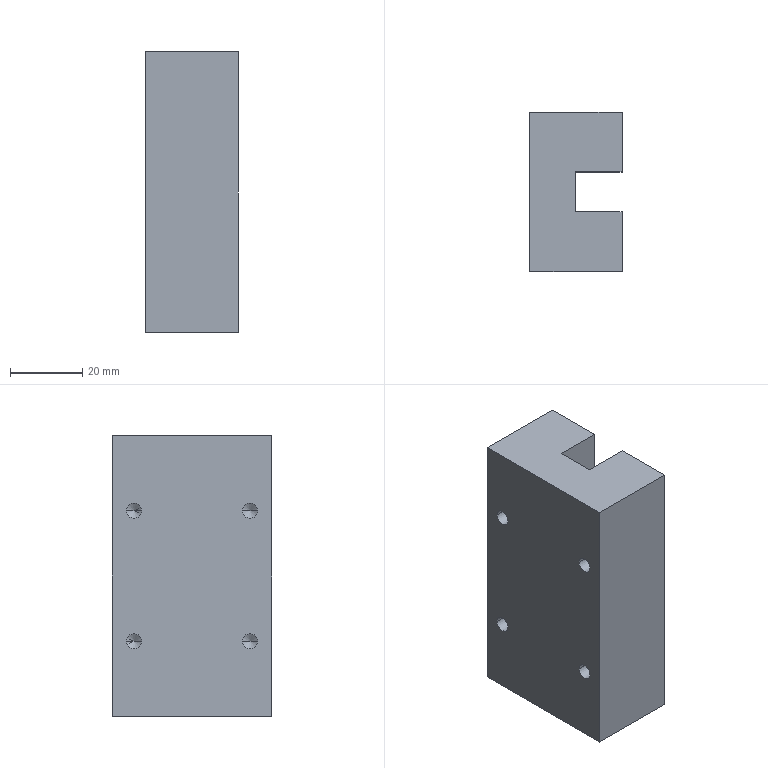Component | SolidWorks | HGH20CASlider-2 | 1 solid | 26 faces | box 25.41 x 44 x 77.5 mm | volume 75261 mm3 | plane 10 | cylinder 8 | cone 8 | commonest cylinder face diameters 4.2 x8
build123d program:
from build123d import *

# Parameters (mm, degrees)
SKETCH1_W             = 44
SKETCH1_H             = 77.5
BOSS_EXTRUDE1_DEPTH   = 25.4
SKETCH2_W             = 11
SKETCH2_H             = 12.9
CUT_EXTRUDE1_DEPTH    = 77.5
M5_TAPPED_HOLE1_D     = 4.2
M5_TAPPED_HOLE1_DEPTH = 6
M5_TAPPED_HOLE1_TIP   = 1.262


with BuildPart() as part:
    # Sketch1 → Boss-Extrude1 (new body)
    with BuildSketch(Plane.XY):
        Rectangle(SKETCH1_W, SKETCH1_H)
    extrude(amount=BOSS_EXTRUDE1_DEPTH)

    # Sketch2 → Cut-Extrude1 (cut)
    with BuildSketch(Plane(origin=(0, 38.75, 0), x_dir=(1, 0, 0), z_dir=(0, 1, 0))):
        with Locations((0, -18.95)):
            Rectangle(SKETCH2_W, SKETCH2_H)
    extrude(amount=-CUT_EXTRUDE1_DEPTH, mode=Mode.SUBTRACT)

    # M5 Tapped Hole1
    with Locations(Plane(origin=(0, 0, 0), x_dir=(-1, 0, 0), z_dir=(0, 0, -1))):
        with Locations((-16, 18), (-16, -18), (16, 18), (16, -18)):
            Hole(M5_TAPPED_HOLE1_D / 2, depth=M5_TAPPED_HOLE1_DEPTH)
            with Locations((0, 0, -(M5_TAPPED_HOLE1_DEPTH + M5_TAPPED_HOLE1_TIP / 2))):  # 118° drill point
                Cone(0, M5_TAPPED_HOLE1_D / 2, M5_TAPPED_HOLE1_TIP, mode=Mode.SUBTRACT)


solid = part.part

# Placed as in the assembly
solid = solid.moved(Location((1956.163, 3833.761, 1079.241), (90, 90, 0)))
STEP:
#1=COLOUR_RGB('',0.7922,0.8196,0.9333);
#2=FILL_AREA_STYLE_COLOUR('',#1);
#3=FILL_AREA_STYLE('',(#2));
#4=SURFACE_STYLE_FILL_AREA(#3);
#5=SURFACE_SIDE_STYLE('',(#4));
#6=SURFACE_STYLE_USAGE(.BOTH.,#5);
#7=PRESENTATION_STYLE_ASSIGNMENT((#6));
#8=CARTESIAN_POINT('',(77.251,150.223,41.781));
#9=VERTEX_POINT('',#8);
#10=CARTESIAN_POINT('',(77.251,150.388,41.781));
#11=VERTEX_POINT('',#10);
#12=CARTESIAN_POINT('',(77.251,150.306,41.781));
#13=DIRECTION('',(-1.,-0.0001552,-0.));
#14=DIRECTION('',(-0.0001552,1.,0.));
#15=AXIS2_PLACEMENT_3D('',#12,#13,#14);
#16=CIRCLE('',#15,0.08268);
#17=EDGE_CURVE('',#9,#11,#16,.T.);
#18=ORIENTED_EDGE('',*,*,#17,.F.);
#19=CARTESIAN_POINT('',(77.014,150.223,41.781));
#20=VERTEX_POINT('',#19);
#21=CARTESIAN_POINT('',(77.014,150.223,41.781));
#22=DIRECTION('',(-1.,-0.0001552,-0.));
#23=VECTOR('',#22,39.37);
#24=LINE('',#21,#23);
#25=EDGE_CURVE('',#9,#20,#24,.T.);
#26=ORIENTED_EDGE('',*,*,#25,.T.);
#27=CARTESIAN_POINT('',(77.014,150.388,41.781));
#28=VERTEX_POINT('',#27);
#29=CARTESIAN_POINT('',(77.014,150.305,41.781));
#30=DIRECTION('',(-1.,-0.0001552,-0.));
#31=DIRECTION('',(-0.0001552,1.,0.));
#32=AXIS2_PLACEMENT_3D('',#29,#30,#31);
#33=CIRCLE('',#32,0.08268);
#34=EDGE_CURVE('',#20,#28,#33,.T.);
#35=ORIENTED_EDGE('',*,*,#34,.T.);
#36=CARTESIAN_POINT('',(77.014,150.388,41.781));
#37=DIRECTION('',(-1.,-0.0001552,-0.));
#38=VECTOR('',#37,39.37);
#39=LINE('',#36,#38);
#40=EDGE_CURVE('',#11,#28,#39,.T.);
#41=ORIENTED_EDGE('',*,*,#40,.F.);
#42=EDGE_LOOP('',(#18,#26,#35,#41));
#43=FACE_OUTER_BOUND('',#42,.T.);
#44=CARTESIAN_POINT('',(77.014,150.305,41.781));
#45=DIRECTION('',(-1.,-0.0001552,-0.));
#46=DIRECTION('',(-0.0001552,1.,0.));
#47=AXIS2_PLACEMENT_3D('',#44,#45,#46);
#48=CYLINDRICAL_SURFACE('',#47,0.08268);
#49=ADVANCED_FACE('',(#43),#48,.F.);
#50=CARTESIAN_POINT('',(77.3,150.306,41.781));
#51=VERTEX_POINT('',#50);
#52=CARTESIAN_POINT('',(77.251,150.388,41.781));
#53=DIRECTION('',(-0.5152,0.8571,-0.));
#54=VECTOR('',#53,39.37);
#55=LINE('',#52,#54);
#56=EDGE_CURVE('',#51,#11,#55,.T.);
#57=ORIENTED_EDGE('',*,*,#56,.F.);
#58=CARTESIAN_POINT('',(77.251,150.223,41.781));
#59=DIRECTION('',(-0.5149,-0.8572,0.));
#60=VECTOR('',#59,39.37);
#61=LINE('',#58,#60);
#62=EDGE_CURVE('',#51,#9,#61,.T.);
#63=ORIENTED_EDGE('',*,*,#62,.T.);
#64=ORIENTED_EDGE('',*,*,#17,.T.);
#65=EDGE_LOOP('',(#57,#63,#64));
#66=FACE_OUTER_BOUND('',#65,.T.);
#67=CARTESIAN_POINT('',(77.251,150.306,41.781));
#68=DIRECTION('',(-1.,-0.0001552,-0.));
#69=DIRECTION('',(-0.0001552,1.,0.));
#70=AXIS2_PLACEMENT_3D('',#67,#68,#69);
#71=CONICAL_SURFACE('',#70,0.08268,1.03);
#72=ADVANCED_FACE('',(#66),#71,.F.);
#73=CARTESIAN_POINT('',(77.251,150.223,43.198));
#74=VERTEX_POINT('',#73);
#75=CARTESIAN_POINT('',(77.251,150.388,43.198));
#76=VERTEX_POINT('',#75);
#77=CARTESIAN_POINT('',(77.251,150.306,43.198));
#78=DIRECTION('',(-1.,-0.0001552,-0.));
#79=DIRECTION('',(-0.0001552,1.,0.));
#80=AXIS2_PLACEMENT_3D('',#77,#78,#79);
#81=CIRCLE('',#80,0.08268);
#82=EDGE_CURVE('',#74,#76,#81,.T.);
#83=ORIENTED_EDGE('',*,*,#82,.F.);
#84=CARTESIAN_POINT('',(77.014,150.223,43.198));
#85=VERTEX_POINT('',#84);
#86=CARTESIAN_POINT('',(77.014,150.223,43.198));
#87=DIRECTION('',(-1.,-0.0001552,-0.));
#88=VECTOR('',#87,39.37);
#89=LINE('',#86,#88);
#90=EDGE_CURVE('',#74,#85,#89,.T.);
#91=ORIENTED_EDGE('',*,*,#90,.T.);
#92=CARTESIAN_POINT('',(77.014,150.388,43.198));
#93=VERTEX_POINT('',#92);
#94=CARTESIAN_POINT('',(77.014,150.305,43.198));
#95=DIRECTION('',(-1.,-0.0001552,-0.));
#96=DIRECTION('',(-0.0001552,1.,0.));
#97=AXIS2_PLACEMENT_3D('',#94,#95,#96);
#98=CIRCLE('',#97,0.08268);
#99=EDGE_CURVE('',#85,#93,#98,.T.);
#100=ORIENTED_EDGE('',*,*,#99,.T.);
#101=CARTESIAN_POINT('',(77.014,150.388,43.198));
#102=DIRECTION('',(-1.,-0.0001552,-0.));
#103=VECTOR('',#102,39.37);
#104=LINE('',#101,#103);
#105=EDGE_CURVE('',#76,#93,#104,.T.);
#106=ORIENTED_EDGE('',*,*,#105,.F.);
#107=EDGE_LOOP('',(#83,#91,#100,#106));
#108=FACE_OUTER_BOUND('',#107,.T.);
#109=CARTESIAN_POINT('',(77.014,150.305,43.198));
#110=DIRECTION('',(-1.,-0.0001552,-0.));
#111=DIRECTION('',(-0.0001552,1.,0.));
#112=AXIS2_PLACEMENT_3D('',#109,#110,#111);
#113=CYLINDRICAL_SURFACE('',#112,0.08268);
#114=ADVANCED_FACE('',(#108),#113,.F.);
#115=CARTESIAN_POINT('',(77.3,150.306,43.198));
#116=VERTEX_POINT('',#115);
#117=CARTESIAN_POINT('',(77.251,150.388,43.198));
#118=DIRECTION('',(-0.5152,0.8571,-0.));
#119=VECTOR('',#118,39.37);
#120=LINE('',#117,#119);
#121=EDGE_CURVE('',#116,#76,#120,.T.);
#122=ORIENTED_EDGE('',*,*,#121,.F.);
#123=CARTESIAN_POINT('',(77.251,150.223,43.198));
#124=DIRECTION('',(-0.5149,-0.8572,0.));
#125=VECTOR('',#124,39.37);
#126=LINE('',#123,#125);
#127=EDGE_CURVE('',#116,#74,#126,.T.);
#128=ORIENTED_EDGE('',*,*,#127,.T.);
#129=ORIENTED_EDGE('',*,*,#82,.T.);
#130=EDGE_LOOP('',(#122,#128,#129));
#131=FACE_OUTER_BOUND('',#130,.T.);
#132=CARTESIAN_POINT('',(77.251,150.306,43.198));
#133=DIRECTION('',(-1.,-0.0001552,-0.));
#134=DIRECTION('',(-0.0001552,1.,0.));
#135=AXIS2_PLACEMENT_3D('',#132,#133,#134);
#136=CONICAL_SURFACE('',#135,0.08268,1.03);
#137=ADVANCED_FACE('',(#131),#136,.F.);
#138=CARTESIAN_POINT('',(77.25,151.483,41.781));
#139=VERTEX_POINT('',#138);
#140=CARTESIAN_POINT('',(77.25,151.648,41.781));
#141=VERTEX_POINT('',#140);
#142=CARTESIAN_POINT('',(77.25,151.565,41.781));
#143=DIRECTION('',(-1.,-0.0001552,-0.));
#144=DIRECTION('',(-0.0001552,1.,0.));
#145=AXIS2_PLACEMENT_3D('',#142,#143,#144);
#146=CIRCLE('',#145,0.08268);
#147=EDGE_CURVE('',#139,#141,#146,.T.);
#148=ORIENTED_EDGE('',*,*,#147,.F.);
#149=CARTESIAN_POINT('',(77.014,151.483,41.781));
#150=VERTEX_POINT('',#149);
#151=CARTESIAN_POINT('',(77.014,151.483,41.781));
#152=DIRECTION('',(-1.,-0.0001552,-0.));
#153=VECTOR('',#152,39.37);
#154=LINE('',#151,#153);
#155=EDGE_CURVE('',#139,#150,#154,.T.);
#156=ORIENTED_EDGE('',*,*,#155,.T.);
#157=CARTESIAN_POINT('',(77.014,151.648,41.781));
#158=VERTEX_POINT('',#157);
#159=CARTESIAN_POINT('',(77.014,151.565,41.781));
#160=DIRECTION('',(-1.,-0.0001552,-0.));
#161=DIRECTION('',(-0.0001552,1.,0.));
#162=AXIS2_PLACEMENT_3D('',#159,#160,#161);
#163=CIRCLE('',#162,0.08268);
#164=EDGE_CURVE('',#150,#158,#163,.T.);
#165=ORIENTED_EDGE('',*,*,#164,.T.);
#166=CARTESIAN_POINT('',(77.014,151.648,41.781));
#167=DIRECTION('',(-1.,-0.0001552,-0.));
#168=VECTOR('',#167,39.37);
#169=LINE('',#166,#168);
#170=EDGE_CURVE('',#141,#158,#169,.T.);
#171=ORIENTED_EDGE('',*,*,#170,.F.);
#172=EDGE_LOOP('',(#148,#156,#165,#171));
#173=FACE_OUTER_BOUND('',#172,.T.);
#174=CARTESIAN_POINT('',(77.014,151.565,41.781));
#175=DIRECTION('',(-1.,-0.0001552,-0.));
#176=DIRECTION('',(-0.0001552,1.,0.));
#177=AXIS2_PLACEMENT_3D('',#174,#175,#176);
#178=CYLINDRICAL_SURFACE('',#177,0.08268);
#179=ADVANCED_FACE('',(#173),#178,.F.);
#180=CARTESIAN_POINT('',(77.3,151.565,41.781));
#181=VERTEX_POINT('',#180);
#182=CARTESIAN_POINT('',(77.25,151.648,41.781));
#183=DIRECTION('',(-0.5152,0.8571,-0.));
#184=VECTOR('',#183,39.37);
#185=LINE('',#182,#184);
#186=EDGE_CURVE('',#181,#141,#185,.T.);
#187=ORIENTED_EDGE('',*,*,#186,.F.);
#188=CARTESIAN_POINT('',(77.25,151.483,41.781));
#189=DIRECTION('',(-0.5149,-0.8572,0.));
#190=VECTOR('',#189,39.37);
#191=LINE('',#188,#190);
#192=EDGE_CURVE('',#181,#139,#191,.T.);
#193=ORIENTED_EDGE('',*,*,#192,.T.);
#194=ORIENTED_EDGE('',*,*,#147,.T.);
#195=EDGE_LOOP('',(#187,#193,#194));
#196=FACE_OUTER_BOUND('',#195,.T.);
#197=CARTESIAN_POINT('',(77.25,151.565,41.781));
#198=DIRECTION('',(-1.,-0.0001552,-0.));
#199=DIRECTION('',(-0.0001552,1.,0.));
#200=AXIS2_PLACEMENT_3D('',#197,#198,#199);
#201=CONICAL_SURFACE('',#200,0.08268,1.03);
#202=ADVANCED_FACE('',(#196),#201,.F.);
#203=CARTESIAN_POINT('',(77.25,151.483,43.198));
#204=VERTEX_POINT('',#203);
#205=CARTESIAN_POINT('',(77.25,151.648,43.198));
#206=VERTEX_POINT('',#205);
#207=CARTESIAN_POINT('',(77.25,151.565,43.198));
#208=DIRECTION('',(-1.,-0.0001552,-0.));
#209=DIRECTION('',(-0.0001552,1.,0.));
#210=AXIS2_PLACEMENT_3D('',#207,#208,#209);
#211=CIRCLE('',#210,0.08268);
#212=EDGE_CURVE('',#204,#206,#211,.T.);
#213=ORIENTED_EDGE('',*,*,#212,.F.);
#214=CARTESIAN_POINT('',(77.014,151.483,43.198));
#215=VERTEX_POINT('',#214);
#216=CARTESIAN_POINT('',(77.014,151.483,43.198));
#217=DIRECTION('',(-1.,-0.0001552,-0.));
#218=VECTOR('',#217,39.37);
#219=LINE('',#216,#218);
#220=EDGE_CURVE('',#204,#215,#219,.T.);
#221=ORIENTED_EDGE('',*,*,#220,.T.);
#222=CARTESIAN_POINT('',(77.014,151.648,43.198));
#223=VERTEX_POINT('',#222);
#224=CARTESIAN_POINT('',(77.014,151.565,43.198));
#225=DIRECTION('',(-1.,-0.0001552,-0.));
#226=DIRECTION('',(-0.0001552,1.,0.));
#227=AXIS2_PLACEMENT_3D('',#224,#225,#226);
#228=CIRCLE('',#227,0.08268);
#229=EDGE_CURVE('',#215,#223,#228,.T.);
#230=ORIENTED_EDGE('',*,*,#229,.T.);
#231=CARTESIAN_POINT('',(77.014,151.648,43.198));
#232=DIRECTION('',(-1.,-0.0001552,-0.));
#233=VECTOR('',#232,39.37);
#234=LINE('',#231,#233);
#235=EDGE_CURVE('',#206,#223,#234,.T.);
#236=ORIENTED_EDGE('',*,*,#235,.F.);
#237=EDGE_LOOP('',(#213,#221,#230,#236));
#238=FACE_OUTER_BOUND('',#237,.T.);
#239=CARTESIAN_POINT('',(77.014,151.565,43.198));
#240=DIRECTION('',(-1.,-0.0001552,-0.));
#241=DIRECTION('',(-0.0001552,1.,0.));
#242=AXIS2_PLACEMENT_3D('',#239,#240,#241);
#243=CYLINDRICAL_SURFACE('',#242,0.08268);
#244=ADVANCED_FACE('',(#238),#243,.F.);
#245=CARTESIAN_POINT('',(77.3,151.565,43.198));
#246=VERTEX_POINT('',#245);
#247=CARTESIAN_POINT('',(77.25,151.648,43.198));
#248=DIRECTION('',(-0.5152,0.8571,-0.));
#249=VECTOR('',#248,39.37);
#250=LINE('',#247,#249);
#251=EDGE_CURVE('',#246,#206,#250,.T.);
#252=ORIENTED_EDGE('',*,*,#251,.F.);
#253=CARTESIAN_POINT('',(77.25,151.483,43.198));
#254=DIRECTION('',(-0.5149,-0.8572,0.));
#255=VECTOR('',#254,39.37);
#256=LINE('',#253,#255);
#257=EDGE_CURVE('',#246,#204,#256,.T.);
#258=ORIENTED_EDGE('',*,*,#257,.T.);
#259=ORIENTED_EDGE('',*,*,#212,.T.);
#260=EDGE_LOOP('',(#252,#258,#259));
#261=FACE_OUTER_BOUND('',#260,.T.);
#262=CARTESIAN_POINT('',(77.25,151.565,43.198));
#263=DIRECTION('',(-1.,-0.0001552,-0.));
#264=DIRECTION('',(-0.0001552,1.,0.));
#265=AXIS2_PLACEMENT_3D('',#262,#263,#264);
#266=CONICAL_SURFACE('',#265,0.08268,1.03);
#267=ADVANCED_FACE('',(#261),#266,.F.);
#268=CARTESIAN_POINT('',(78.014,151.152,44.015));
#269=VERTEX_POINT('',#268);
#270=CARTESIAN_POINT('',(78.014,151.152,40.964));
#271=VERTEX_POINT('',#270);
#272=CARTESIAN_POINT('',(78.014,151.152,44.683));
#273=DIRECTION('',(0.,-0.,-1.));
#274=VECTOR('',#273,39.37);
#275=LINE('',#272,#274);
#276=EDGE_CURVE('',#269,#271,#275,.T.);
#277=ORIENTED_EDGE('',*,*,#276,.T.);
#278=CARTESIAN_POINT('',(78.014,151.802,40.964));
#279=VERTEX_POINT('',#278);
#280=CARTESIAN_POINT('',(78.014,150.069,40.964));
#281=DIRECTION('',(-0.0001552,1.,-0.));
#282=VECTOR('',#281,39.37);
#283=LINE('',#280,#282);
#284=EDGE_CURVE('',#271,#279,#283,.T.);
#285=ORIENTED_EDGE('',*,*,#284,.T.);
#286=CARTESIAN_POINT('',(78.014,151.802,44.015));
#287=VERTEX_POINT('',#286);
#288=CARTESIAN_POINT('',(78.014,151.802,44.015));
#289=DIRECTION('',(-0.,0.,1.));
#290=VECTOR('',#289,39.37);
#291=LINE('',#288,#290);
#292=EDGE_CURVE('',#279,#287,#291,.T.);
#293=ORIENTED_EDGE('',*,*,#292,.T.);
#294=CARTESIAN_POINT('',(78.014,150.069,44.015));
#295=DIRECTION('',(0.0001552,-1.,0.));
#296=VECTOR('',#295,39.37);
#297=LINE('',#294,#296);
#298=EDGE_CURVE('',#287,#269,#297,.T.);
#299=ORIENTED_EDGE('',*,*,#298,.T.);
#300=EDGE_LOOP('',(#277,#285,#293,#299));
#301=FACE_OUTER_BOUND('',#300,.T.);
#302=CARTESIAN_POINT('',(78.014,150.936,42.49));
#303=DIRECTION('',(1.,0.0001552,0.));
#304=DIRECTION('',(0.0001552,-1.,0.));
#305=AXIS2_PLACEMENT_3D('',#302,#303,#304);
#306=PLANE('',#305);
#307=ADVANCED_FACE('',(#301),#306,.T.);
#308=CARTESIAN_POINT('',(77.014,151.802,40.964));
#309=VERTEX_POINT('',#308);
#310=CARTESIAN_POINT('',(77.014,151.802,44.015));
#311=VERTEX_POINT('',#310);
#312=CARTESIAN_POINT('',(77.014,151.802,44.015));
#313=DIRECTION('',(-0.,0.,1.));
#314=VECTOR('',#313,39.37);
#315=LINE('',#312,#314);
#316=EDGE_CURVE('',#309,#311,#315,.T.);
#317=ORIENTED_EDGE('',*,*,#316,.T.);
#318=CARTESIAN_POINT('',(78.014,151.802,44.015));
#319=DIRECTION('',(-1.,-0.0001552,-0.));
#320=VECTOR('',#319,39.37);
#321=LINE('',#318,#320);
#322=EDGE_CURVE('',#287,#311,#321,.T.);
#323=ORIENTED_EDGE('',*,*,#322,.F.);
#324=ORIENTED_EDGE('',*,*,#292,.F.);
#325=CARTESIAN_POINT('',(78.014,151.802,40.964));
#326=DIRECTION('',(-1.,-0.0001552,-0.));
#327=VECTOR('',#326,39.37);
#328=LINE('',#325,#327);
#329=EDGE_CURVE('',#279,#309,#328,.T.);
#330=ORIENTED_EDGE('',*,*,#329,.T.);
#331=EDGE_LOOP('',(#317,#323,#324,#330));
#332=FACE_OUTER_BOUND('',#331,.T.);
#333=CARTESIAN_POINT('',(78.014,151.802,44.015));
#334=DIRECTION('',(0.0001552,-1.,0.));
#335=DIRECTION('',(-1.,-0.0001552,-0.));
#336=AXIS2_PLACEMENT_3D('',#333,#334,#335);
#337=PLANE('',#336);
#338=ADVANCED_FACE('',(#332),#337,.F.);
#339=CARTESIAN_POINT('',(77.506,151.152,44.015));
#340=VERTEX_POINT('',#339);
#341=CARTESIAN_POINT('',(77.506,150.719,44.015));
#342=VERTEX_POINT('',#341);
#343=CARTESIAN_POINT('',(77.506,151.152,44.015));
#344=DIRECTION('',(0.0001552,-1.,0.));
#345=VECTOR('',#344,39.37);
#346=LINE('',#343,#345);
#347=EDGE_CURVE('',#340,#342,#346,.T.);
#348=ORIENTED_EDGE('',*,*,#347,.F.);
#349=CARTESIAN_POINT('',(78.014,151.152,44.015));
#350=DIRECTION('',(-1.,-0.0001552,-0.));
#351=VECTOR('',#350,39.37);
#352=LINE('',#349,#351);
#353=EDGE_CURVE('',#269,#340,#352,.T.);
#354=ORIENTED_EDGE('',*,*,#353,.F.);
#355=ORIENTED_EDGE('',*,*,#298,.F.);
#356=ORIENTED_EDGE('',*,*,#322,.T.);
#357=CARTESIAN_POINT('',(77.014,150.069,44.015));
#358=VERTEX_POINT('',#357);
#359=CARTESIAN_POINT('',(77.014,150.069,44.015));
#360=DIRECTION('',(0.0001552,-1.,0.));
#361=VECTOR('',#360,39.37);
#362=LINE('',#359,#361);
#363=EDGE_CURVE('',#311,#358,#362,.T.);
#364=ORIENTED_EDGE('',*,*,#363,.T.);
#365=CARTESIAN_POINT('',(78.014,150.069,44.015));
#366=VERTEX_POINT('',#365);
#367=CARTESIAN_POINT('',(78.014,150.069,44.015));
#368=DIRECTION('',(-1.,-0.0001552,-0.));
#369=VECTOR('',#368,39.37);
#370=LINE('',#367,#369);
#371=EDGE_CURVE('',#366,#358,#370,.T.);
#372=ORIENTED_EDGE('',*,*,#371,.F.);
#373=CARTESIAN_POINT('',(78.014,150.719,44.015));
#374=VERTEX_POINT('',#373);
#375=CARTESIAN_POINT('',(78.014,150.069,44.015));
#376=DIRECTION('',(0.0001552,-1.,0.));
#377=VECTOR('',#376,39.37);
#378=LINE('',#375,#377);
#379=EDGE_CURVE('',#374,#366,#378,.T.);
#380=ORIENTED_EDGE('',*,*,#379,.F.);
#381=CARTESIAN_POINT('',(78.014,150.719,44.015));
#382=DIRECTION('',(1.,0.0001552,0.));
#383=VECTOR('',#382,39.37);
#384=LINE('',#381,#383);
#385=EDGE_CURVE('',#342,#374,#384,.T.);
#386=ORIENTED_EDGE('',*,*,#385,.F.);
#387=EDGE_LOOP('',(#348,#354,#355,#356,#364,#372,#380,#386));
#388=FACE_OUTER_BOUND('',#387,.T.);
#389=CARTESIAN_POINT('',(78.014,150.069,44.015));
#390=DIRECTION('',(0.,-0.,-1.));
#391=DIRECTION('',(1.,0.0001552,0.));
#392=AXIS2_PLACEMENT_3D('',#389,#390,#391);
#393=PLANE('',#392);
#394=ADVANCED_FACE('',(#388),#393,.F.);
#395=CARTESIAN_POINT('',(77.014,150.069,40.964));
#396=VERTEX_POINT('',#395);
#397=CARTESIAN_POINT('',(77.014,150.069,44.015));
#398=DIRECTION('',(0.,-0.,-1.));
#399=VECTOR('',#398,39.37);
#400=LINE('',#397,#399);
#401=EDGE_CURVE('',#358,#396,#400,.T.);
#402=ORIENTED_EDGE('',*,*,#401,.T.);
#403=CARTESIAN_POINT('',(78.014,150.069,40.964));
#404=VERTEX_POINT('',#403);
#405=CARTESIAN_POINT('',(78.014,150.069,40.964));
#406=DIRECTION('',(-1.,-0.0001552,-0.));
#407=VECTOR('',#406,39.37);
#408=LINE('',#405,#407);
#409=EDGE_CURVE('',#404,#396,#408,.T.);
#410=ORIENTED_EDGE('',*,*,#409,.F.);
#411=CARTESIAN_POINT('',(78.014,150.069,44.015));
#412=DIRECTION('',(0.,-0.,-1.));
#413=VECTOR('',#412,39.37);
#414=LINE('',#411,#413);
#415=EDGE_CURVE('',#366,#404,#414,.T.);
#416=ORIENTED_EDGE('',*,*,#415,.F.);
#417=ORIENTED_EDGE('',*,*,#371,.T.);
#418=EDGE_LOOP('',(#402,#410,#416,#417));
#419=FACE_OUTER_BOUND('',#418,.T.);
#420=CARTESIAN_POINT('',(78.014,150.069,44.015));
#421=DIRECTION('',(-0.0001552,1.,-0.));
#422=DIRECTION('',(1.,0.0001552,0.));
#423=AXIS2_PLACEMENT_3D('',#420,#421,#422);
#424=PLANE('',#423);
#425=ADVANCED_FACE('',(#419),#424,.F.);
#426=ORIENTED_EDGE('',*,*,#284,.F.);
#427=CARTESIAN_POINT('',(77.506,151.152,40.964));
#428=VERTEX_POINT('',#427);
#429=CARTESIAN_POINT('',(78.014,151.152,40.964));
#430=DIRECTION('',(1.,0.0001552,0.));
#431=VECTOR('',#430,39.37);
#432=LINE('',#429,#431);
#433=EDGE_CURVE('',#428,#271,#432,.T.);
#434=ORIENTED_EDGE('',*,*,#433,.F.);
#435=CARTESIAN_POINT('',(77.506,150.719,40.964));
#436=VERTEX_POINT('',#435);
#437=CARTESIAN_POINT('',(77.506,151.152,40.964));
#438=DIRECTION('',(-0.0001552,1.,-0.));
#439=VECTOR('',#438,39.37);
#440=LINE('',#437,#439);
#441=EDGE_CURVE('',#436,#428,#440,.T.);
#442=ORIENTED_EDGE('',*,*,#441,.F.);
#443=CARTESIAN_POINT('',(78.014,150.719,40.964));
#444=VERTEX_POINT('',#443);
#445=CARTESIAN_POINT('',(78.014,150.719,40.964));
#446=DIRECTION('',(-1.,-0.0001552,-0.));
#447=VECTOR('',#446,39.37);
#448=LINE('',#445,#447);
#449=EDGE_CURVE('',#444,#436,#448,.T.);
#450=ORIENTED_EDGE('',*,*,#449,.F.);
#451=CARTESIAN_POINT('',(78.014,150.069,40.964));
#452=DIRECTION('',(-0.0001552,1.,-0.));
#453=VECTOR('',#452,39.37);
#454=LINE('',#451,#453);
#455=EDGE_CURVE('',#404,#444,#454,.T.);
#456=ORIENTED_EDGE('',*,*,#455,.F.);
#457=ORIENTED_EDGE('',*,*,#409,.T.);
#458=CARTESIAN_POINT('',(77.014,150.069,40.964));
#459=DIRECTION('',(-0.0001552,1.,-0.));
#460=VECTOR('',#459,39.37);
#461=LINE('',#458,#460);
#462=EDGE_CURVE('',#396,#309,#461,.T.);
#463=ORIENTED_EDGE('',*,*,#462,.T.);
#464=ORIENTED_EDGE('',*,*,#329,.F.);
#465=EDGE_LOOP('',(#426,#434,#442,#450,#456,#457,#463,#464));
#466=FACE_OUTER_BOUND('',#465,.T.);
#467=CARTESIAN_POINT('',(78.014,150.069,40.964));
#468=DIRECTION('',(-0.,0.,1.));
#469=DIRECTION('',(0.0001552,-1.,0.));
#470=AXIS2_PLACEMENT_3D('',#467,#468,#469);
#471=PLANE('',#470);
#472=ADVANCED_FACE('',(#466),#471,.F.);
#473=CARTESIAN_POINT('',(78.014,150.719,44.683));
#474=DIRECTION('',(0.,-0.,-1.));
#475=VECTOR('',#474,39.37);
#476=LINE('',#473,#475);
#477=EDGE_CURVE('',#374,#444,#476,.T.);
#478=ORIENTED_EDGE('',*,*,#477,.F.);
#479=ORIENTED_EDGE('',*,*,#379,.T.);
#480=ORIENTED_EDGE('',*,*,#415,.T.);
#481=ORIENTED_EDGE('',*,*,#455,.T.);
#482=EDGE_LOOP('',(#478,#479,#480,#481));
#483=FACE_OUTER_BOUND('',#482,.T.);
#484=CARTESIAN_POINT('',(78.014,150.936,42.49));
#485=DIRECTION('',(1.,0.0001552,0.));
#486=DIRECTION('',(0.0001552,-1.,0.));
#487=AXIS2_PLACEMENT_3D('',#484,#485,#486);
#488=PLANE('',#487);
#489=ADVANCED_FACE('',(#483),#488,.T.);
#490=CARTESIAN_POINT('',(77.014,150.305,41.781));
#491=DIRECTION('',(-1.,-0.0001552,-0.));
#492=DIRECTION('',(-0.0001552,1.,0.));
#493=AXIS2_PLACEMENT_3D('',#490,#491,#492);
#494=CIRCLE('',#493,0.08268);
#495=EDGE_CURVE('',#28,#20,#494,.T.);
#496=ORIENTED_EDGE('',*,*,#495,.F.);
#497=ORIENTED_EDGE('',*,*,#34,.F.);
#498=EDGE_LOOP('',(#496,#497));
#499=FACE_BOUND('',#498,.T.);
#500=CARTESIAN_POINT('',(77.014,150.305,43.198));
#501=DIRECTION('',(-1.,-0.0001552,-0.));
#502=DIRECTION('',(-0.0001552,1.,0.));
#503=AXIS2_PLACEMENT_3D('',#500,#501,#502);
#504=CIRCLE('',#503,0.08268);
#505=EDGE_CURVE('',#93,#85,#504,.T.);
#506=ORIENTED_EDGE('',*,*,#505,.F.);
#507=ORIENTED_EDGE('',*,*,#99,.F.);
#508=EDGE_LOOP('',(#506,#507));
#509=FACE_BOUND('',#508,.T.);
#510=CARTESIAN_POINT('',(77.014,151.565,41.781));
#511=DIRECTION('',(-1.,-0.0001552,-0.));
#512=DIRECTION('',(-0.0001552,1.,0.));
#513=AXIS2_PLACEMENT_3D('',#510,#511,#512);
#514=CIRCLE('',#513,0.08268);
#515=EDGE_CURVE('',#158,#150,#514,.T.);
#516=ORIENTED_EDGE('',*,*,#515,.F.);
#517=ORIENTED_EDGE('',*,*,#164,.F.);
#518=EDGE_LOOP('',(#516,#517));
#519=FACE_BOUND('',#518,.T.);
#520=CARTESIAN_POINT('',(77.014,151.565,43.198));
#521=DIRECTION('',(-1.,-0.0001552,-0.));
#522=DIRECTION('',(-0.0001552,1.,0.));
#523=AXIS2_PLACEMENT_3D('',#520,#521,#522);
#524=CIRCLE('',#523,0.08268);
#525=EDGE_CURVE('',#223,#215,#524,.T.);
#526=ORIENTED_EDGE('',*,*,#525,.F.);
#527=ORIENTED_EDGE('',*,*,#229,.F.);
#528=EDGE_LOOP('',(#526,#527));
#529=FACE_BOUND('',#528,.T.);
#530=ORIENTED_EDGE('',*,*,#316,.F.);
#531=ORIENTED_EDGE('',*,*,#462,.F.);
#532=ORIENTED_EDGE('',*,*,#401,.F.);
#533=ORIENTED_EDGE('',*,*,#363,.F.);
#534=EDGE_LOOP('',(#530,#531,#532,#533));
#535=FACE_OUTER_BOUND('',#534,.T.);
#536=CARTESIAN_POINT('',(77.014,150.935,42.49));
#537=DIRECTION('',(1.,0.0001552,0.));
#538=DIRECTION('',(0.0001552,-1.,0.));
#539=AXIS2_PLACEMENT_3D('',#536,#537,#538);
#540=PLANE('',#539);
#541=ADVANCED_FACE('',(#499,#509,#519,#529,#535),#540,.F.);
#542=ORIENTED_EDGE('',*,*,#353,.T.);
#543=CARTESIAN_POINT('',(77.506,151.152,44.683));
#544=DIRECTION('',(0.,-0.,-1.));
#545=VECTOR('',#544,39.37);
#546=LINE('',#543,#545);
#547=EDGE_CURVE('',#340,#428,#546,.T.);
#548=ORIENTED_EDGE('',*,*,#547,.T.);
#549=ORIENTED_EDGE('',*,*,#433,.T.);
#550=ORIENTED_EDGE('',*,*,#276,.F.);
#551=EDGE_LOOP('',(#542,#548,#549,#550));
#552=FACE_OUTER_BOUND('',#551,.T.);
#553=CARTESIAN_POINT('',(78.014,151.152,44.683));
#554=DIRECTION('',(-0.0001552,1.,-0.));
#555=DIRECTION('',(-0.,0.,1.));
#556=AXIS2_PLACEMENT_3D('',#553,#554,#555);
#557=PLANE('',#556);
#558=ADVANCED_FACE('',(#552),#557,.F.);
#559=ORIENTED_EDGE('',*,*,#347,.T.);
#560=CARTESIAN_POINT('',(77.506,150.719,44.683));
#561=DIRECTION('',(0.,-0.,-1.));
#562=VECTOR('',#561,39.37);
#563=LINE('',#560,#562);
#564=EDGE_CURVE('',#342,#436,#563,.T.);
#565=ORIENTED_EDGE('',*,*,#564,.T.);
#566=ORIENTED_EDGE('',*,*,#441,.T.);
#567=ORIENTED_EDGE('',*,*,#547,.F.);
#568=EDGE_LOOP('',(#559,#565,#566,#567));
#569=FACE_OUTER_BOUND('',#568,.T.);
#570=CARTESIAN_POINT('',(77.506,151.152,44.683));
#571=DIRECTION('',(-1.,-0.0001552,-0.));
#572=DIRECTION('',(-0.0001552,1.,-0.));
#573=AXIS2_PLACEMENT_3D('',#570,#571,#572);
#574=PLANE('',#573);
#575=ADVANCED_FACE('',(#569),#574,.F.);
#576=ORIENTED_EDGE('',*,*,#385,.T.);
#577=ORIENTED_EDGE('',*,*,#477,.T.);
#578=ORIENTED_EDGE('',*,*,#449,.T.);
#579=ORIENTED_EDGE('',*,*,#564,.F.);
#580=EDGE_LOOP('',(#576,#577,#578,#579));
#581=FACE_OUTER_BOUND('',#580,.T.);
#582=CARTESIAN_POINT('',(78.014,150.719,44.683));
#583=DIRECTION('',(0.0001552,-1.,0.));
#584=DIRECTION('',(-1.,-0.0001552,-0.));
#585=AXIS2_PLACEMENT_3D('',#582,#583,#584);
#586=PLANE('',#585);
#587=ADVANCED_FACE('',(#581),#586,.F.);
#588=ORIENTED_EDGE('',*,*,#257,.F.);
#589=ORIENTED_EDGE('',*,*,#251,.T.);
#590=CARTESIAN_POINT('',(77.25,151.565,43.198));
#591=DIRECTION('',(-1.,-0.0001552,-0.));
#592=DIRECTION('',(-0.0001552,1.,0.));
#593=AXIS2_PLACEMENT_3D('',#590,#591,#592);
#594=CIRCLE('',#593,0.08268);
#595=EDGE_CURVE('',#206,#204,#594,.T.);
#596=ORIENTED_EDGE('',*,*,#595,.T.);
#597=EDGE_LOOP('',(#588,#589,#596));
#598=FACE_OUTER_BOUND('',#597,.T.);
#599=CARTESIAN_POINT('',(77.25,151.565,43.198));
#600=DIRECTION('',(-1.,-0.0001552,-0.));
#601=DIRECTION('',(-0.0001552,1.,0.));
#602=AXIS2_PLACEMENT_3D('',#599,#600,#601);
#603=CONICAL_SURFACE('',#602,0.08268,1.03);
#604=ADVANCED_FACE('',(#598),#603,.F.);
#605=ORIENTED_EDGE('',*,*,#220,.F.);
#606=ORIENTED_EDGE('',*,*,#595,.F.);
#607=ORIENTED_EDGE('',*,*,#235,.T.);
#608=ORIENTED_EDGE('',*,*,#525,.T.);
#609=EDGE_LOOP('',(#605,#606,#607,#608));
#610=FACE_OUTER_BOUND('',#609,.T.);
#611=CARTESIAN_POINT('',(77.014,151.565,43.198));
#612=DIRECTION('',(-1.,-0.0001552,-0.));
#613=DIRECTION('',(-0.0001552,1.,0.));
#614=AXIS2_PLACEMENT_3D('',#611,#612,#613);
#615=CYLINDRICAL_SURFACE('',#614,0.08268);
#616=ADVANCED_FACE('',(#610),#615,.F.);
#617=ORIENTED_EDGE('',*,*,#192,.F.);
#618=ORIENTED_EDGE('',*,*,#186,.T.);
#619=CARTESIAN_POINT('',(77.25,151.565,41.781));
#620=DIRECTION('',(-1.,-0.0001552,-0.));
#621=DIRECTION('',(-0.0001552,1.,0.));
#622=AXIS2_PLACEMENT_3D('',#619,#620,#621);
#623=CIRCLE('',#622,0.08268);
#624=EDGE_CURVE('',#141,#139,#623,.T.);
#625=ORIENTED_EDGE('',*,*,#624,.T.);
#626=EDGE_LOOP('',(#617,#618,#625));
#627=FACE_OUTER_BOUND('',#626,.T.);
#628=CARTESIAN_POINT('',(77.25,151.565,41.781));
#629=DIRECTION('',(-1.,-0.0001552,-0.));
#630=DIRECTION('',(-0.0001552,1.,0.));
#631=AXIS2_PLACEMENT_3D('',#628,#629,#630);
#632=CONICAL_SURFACE('',#631,0.08268,1.03);
#633=ADVANCED_FACE('',(#627),#632,.F.);
#634=ORIENTED_EDGE('',*,*,#155,.F.);
#635=ORIENTED_EDGE('',*,*,#624,.F.);
#636=ORIENTED_EDGE('',*,*,#170,.T.);
#637=ORIENTED_EDGE('',*,*,#515,.T.);
#638=EDGE_LOOP('',(#634,#635,#636,#637));
#639=FACE_OUTER_BOUND('',#638,.T.);
#640=CARTESIAN_POINT('',(77.014,151.565,41.781));
#641=DIRECTION('',(-1.,-0.0001552,-0.));
#642=DIRECTION('',(-0.0001552,1.,0.));
#643=AXIS2_PLACEMENT_3D('',#640,#641,#642);
#644=CYLINDRICAL_SURFACE('',#643,0.08268);
#645=ADVANCED_FACE('',(#639),#644,.F.);
#646=ORIENTED_EDGE('',*,*,#127,.F.);
#647=ORIENTED_EDGE('',*,*,#121,.T.);
#648=CARTESIAN_POINT('',(77.251,150.306,43.198));
#649=DIRECTION('',(-1.,-0.0001552,-0.));
#650=DIRECTION('',(-0.0001552,1.,0.));
#651=AXIS2_PLACEMENT_3D('',#648,#649,#650);
#652=CIRCLE('',#651,0.08268);
#653=EDGE_CURVE('',#76,#74,#652,.T.);
#654=ORIENTED_EDGE('',*,*,#653,.T.);
#655=EDGE_LOOP('',(#646,#647,#654));
#656=FACE_OUTER_BOUND('',#655,.T.);
#657=CARTESIAN_POINT('',(77.251,150.306,43.198));
#658=DIRECTION('',(-1.,-0.0001552,-0.));
#659=DIRECTION('',(-0.0001552,1.,0.));
#660=AXIS2_PLACEMENT_3D('',#657,#658,#659);
#661=CONICAL_SURFACE('',#660,0.08268,1.03);
#662=ADVANCED_FACE('',(#656),#661,.F.);
#663=ORIENTED_EDGE('',*,*,#90,.F.);
#664=ORIENTED_EDGE('',*,*,#653,.F.);
#665=ORIENTED_EDGE('',*,*,#105,.T.);
#666=ORIENTED_EDGE('',*,*,#505,.T.);
#667=EDGE_LOOP('',(#663,#664,#665,#666));
#668=FACE_OUTER_BOUND('',#667,.T.);
#669=CARTESIAN_POINT('',(77.014,150.305,43.198));
#670=DIRECTION('',(-1.,-0.0001552,-0.));
#671=DIRECTION('',(-0.0001552,1.,0.));
#672=AXIS2_PLACEMENT_3D('',#669,#670,#671);
#673=CYLINDRICAL_SURFACE('',#672,0.08268);
#674=ADVANCED_FACE('',(#668),#673,.F.);
#675=ORIENTED_EDGE('',*,*,#62,.F.);
#676=ORIENTED_EDGE('',*,*,#56,.T.);
#677=CARTESIAN_POINT('',(77.251,150.306,41.781));
#678=DIRECTION('',(-1.,-0.0001552,-0.));
#679=DIRECTION('',(-0.0001552,1.,0.));
#680=AXIS2_PLACEMENT_3D('',#677,#678,#679);
#681=CIRCLE('',#680,0.08268);
#682=EDGE_CURVE('',#11,#9,#681,.T.);
#683=ORIENTED_EDGE('',*,*,#682,.T.);
#684=EDGE_LOOP('',(#675,#676,#683));
#685=FACE_OUTER_BOUND('',#684,.T.);
#686=CARTESIAN_POINT('',(77.251,150.306,41.781));
#687=DIRECTION('',(-1.,-0.0001552,-0.));
#688=DIRECTION('',(-0.0001552,1.,0.));
#689=AXIS2_PLACEMENT_3D('',#686,#687,#688);
#690=CONICAL_SURFACE('',#689,0.08268,1.03);
#691=ADVANCED_FACE('',(#685),#690,.F.);
#692=ORIENTED_EDGE('',*,*,#25,.F.);
#693=ORIENTED_EDGE('',*,*,#682,.F.);
#694=ORIENTED_EDGE('',*,*,#40,.T.);
#695=ORIENTED_EDGE('',*,*,#495,.T.);
#696=EDGE_LOOP('',(#692,#693,#694,#695));
#697=FACE_OUTER_BOUND('',#696,.T.);
#698=CARTESIAN_POINT('',(77.014,150.305,41.781));
#699=DIRECTION('',(-1.,-0.0001552,-0.));
#700=DIRECTION('',(-0.0001552,1.,0.));
#701=AXIS2_PLACEMENT_3D('',#698,#699,#700);
#702=CYLINDRICAL_SURFACE('',#701,0.08268);
#703=ADVANCED_FACE('',(#697),#702,.F.);
#704=CLOSED_SHELL('',(#49,#72,#114,#137,#179,#202,#244,#267,#307,#338,#394,#425,#472,#489,#541,#558,#575,#587,#604,#616,#633,#645,#662,#674,#691,#703));
#705=MANIFOLD_SOLID_BREP('',#704);
#706=STYLED_ITEM('',(#7),#705);
#707=(LENGTH_UNIT()NAMED_UNIT(*)SI_UNIT($,.METRE.));
#708=LENGTH_MEASURE_WITH_UNIT(LENGTH_MEASURE(0.0254),#707);
#709=DIMENSIONAL_EXPONENTS(1.,0.,0.,0.,0.,0.,0.);
#710=(CONVERSION_BASED_UNIT('',#708)LENGTH_UNIT()NAMED_UNIT(#709));
#711=UNCERTAINTY_MEASURE_WITH_UNIT(LENGTH_MEASURE(0.00001),#710,'','');
#712=(NAMED_UNIT(*)PLANE_ANGLE_UNIT()SI_UNIT($,.RADIAN.));
#713=(NAMED_UNIT(*)SI_UNIT($,.STERADIAN.)SOLID_ANGLE_UNIT());
#714=(GEOMETRIC_REPRESENTATION_CONTEXT(3)GLOBAL_UNCERTAINTY_ASSIGNED_CONTEXT((#711))GLOBAL_UNIT_ASSIGNED_CONTEXT((#710,#712,#713))REPRESENTATION_CONTEXT('',''));
#715=MECHANICAL_DESIGN_GEOMETRIC_PRESENTATION_REPRESENTATION('',(#706),#714);
#716=CARTESIAN_POINT('',(0.,0.,0.));
#717=DIRECTION('',(0.,0.,1.));
#718=DIRECTION('',(1.,0.,0.));
#719=AXIS2_PLACEMENT_3D('',#716,#717,#718);
#720=(LENGTH_UNIT()NAMED_UNIT(*)SI_UNIT($,.METRE.));
#721=LENGTH_MEASURE_WITH_UNIT(LENGTH_MEASURE(0.0254),#720);
#722=DIMENSIONAL_EXPONENTS(1.,0.,0.,0.,0.,0.,0.);
#723=(CONVERSION_BASED_UNIT('',#721)LENGTH_UNIT()NAMED_UNIT(#722));
#724=UNCERTAINTY_MEASURE_WITH_UNIT(LENGTH_MEASURE(0.00001),#723,'','');
#725=(NAMED_UNIT(*)PLANE_ANGLE_UNIT()SI_UNIT($,.RADIAN.));
#726=(NAMED_UNIT(*)SI_UNIT($,.STERADIAN.)SOLID_ANGLE_UNIT());
#727=(GEOMETRIC_REPRESENTATION_CONTEXT(3)GLOBAL_UNCERTAINTY_ASSIGNED_CONTEXT((#724))GLOBAL_UNIT_ASSIGNED_CONTEXT((#723,#725,#726))REPRESENTATION_CONTEXT('',''));
#728=ADVANCED_BREP_SHAPE_REPRESENTATION('',(#705,#719),#727);
#729=PRESENTATION_LAYER_ASSIGNMENT('','',(#706));